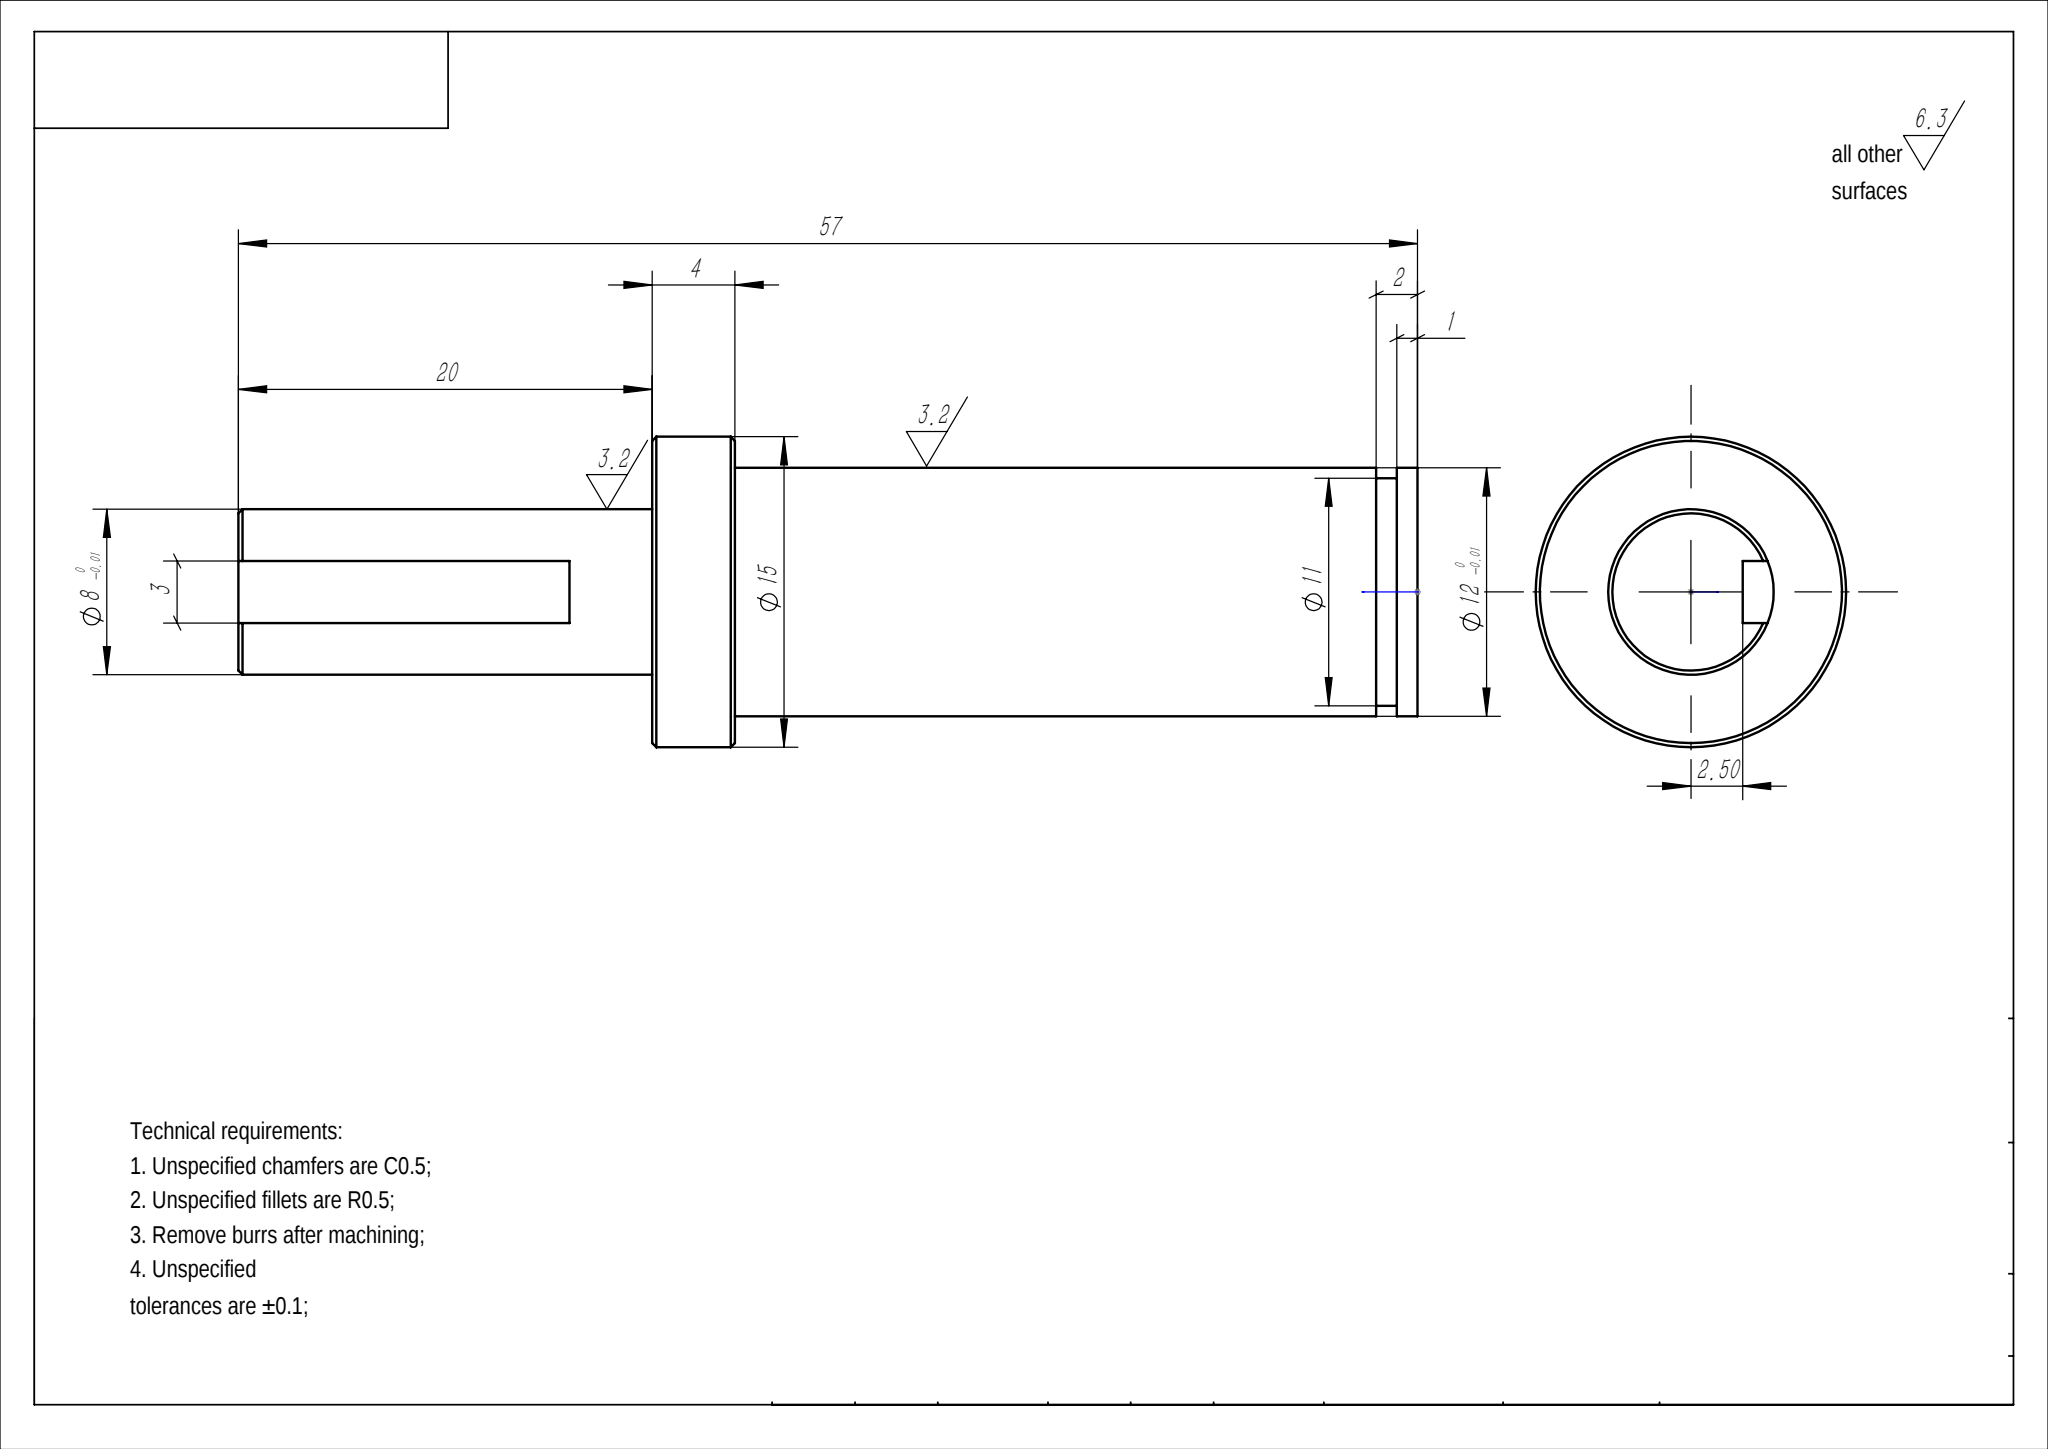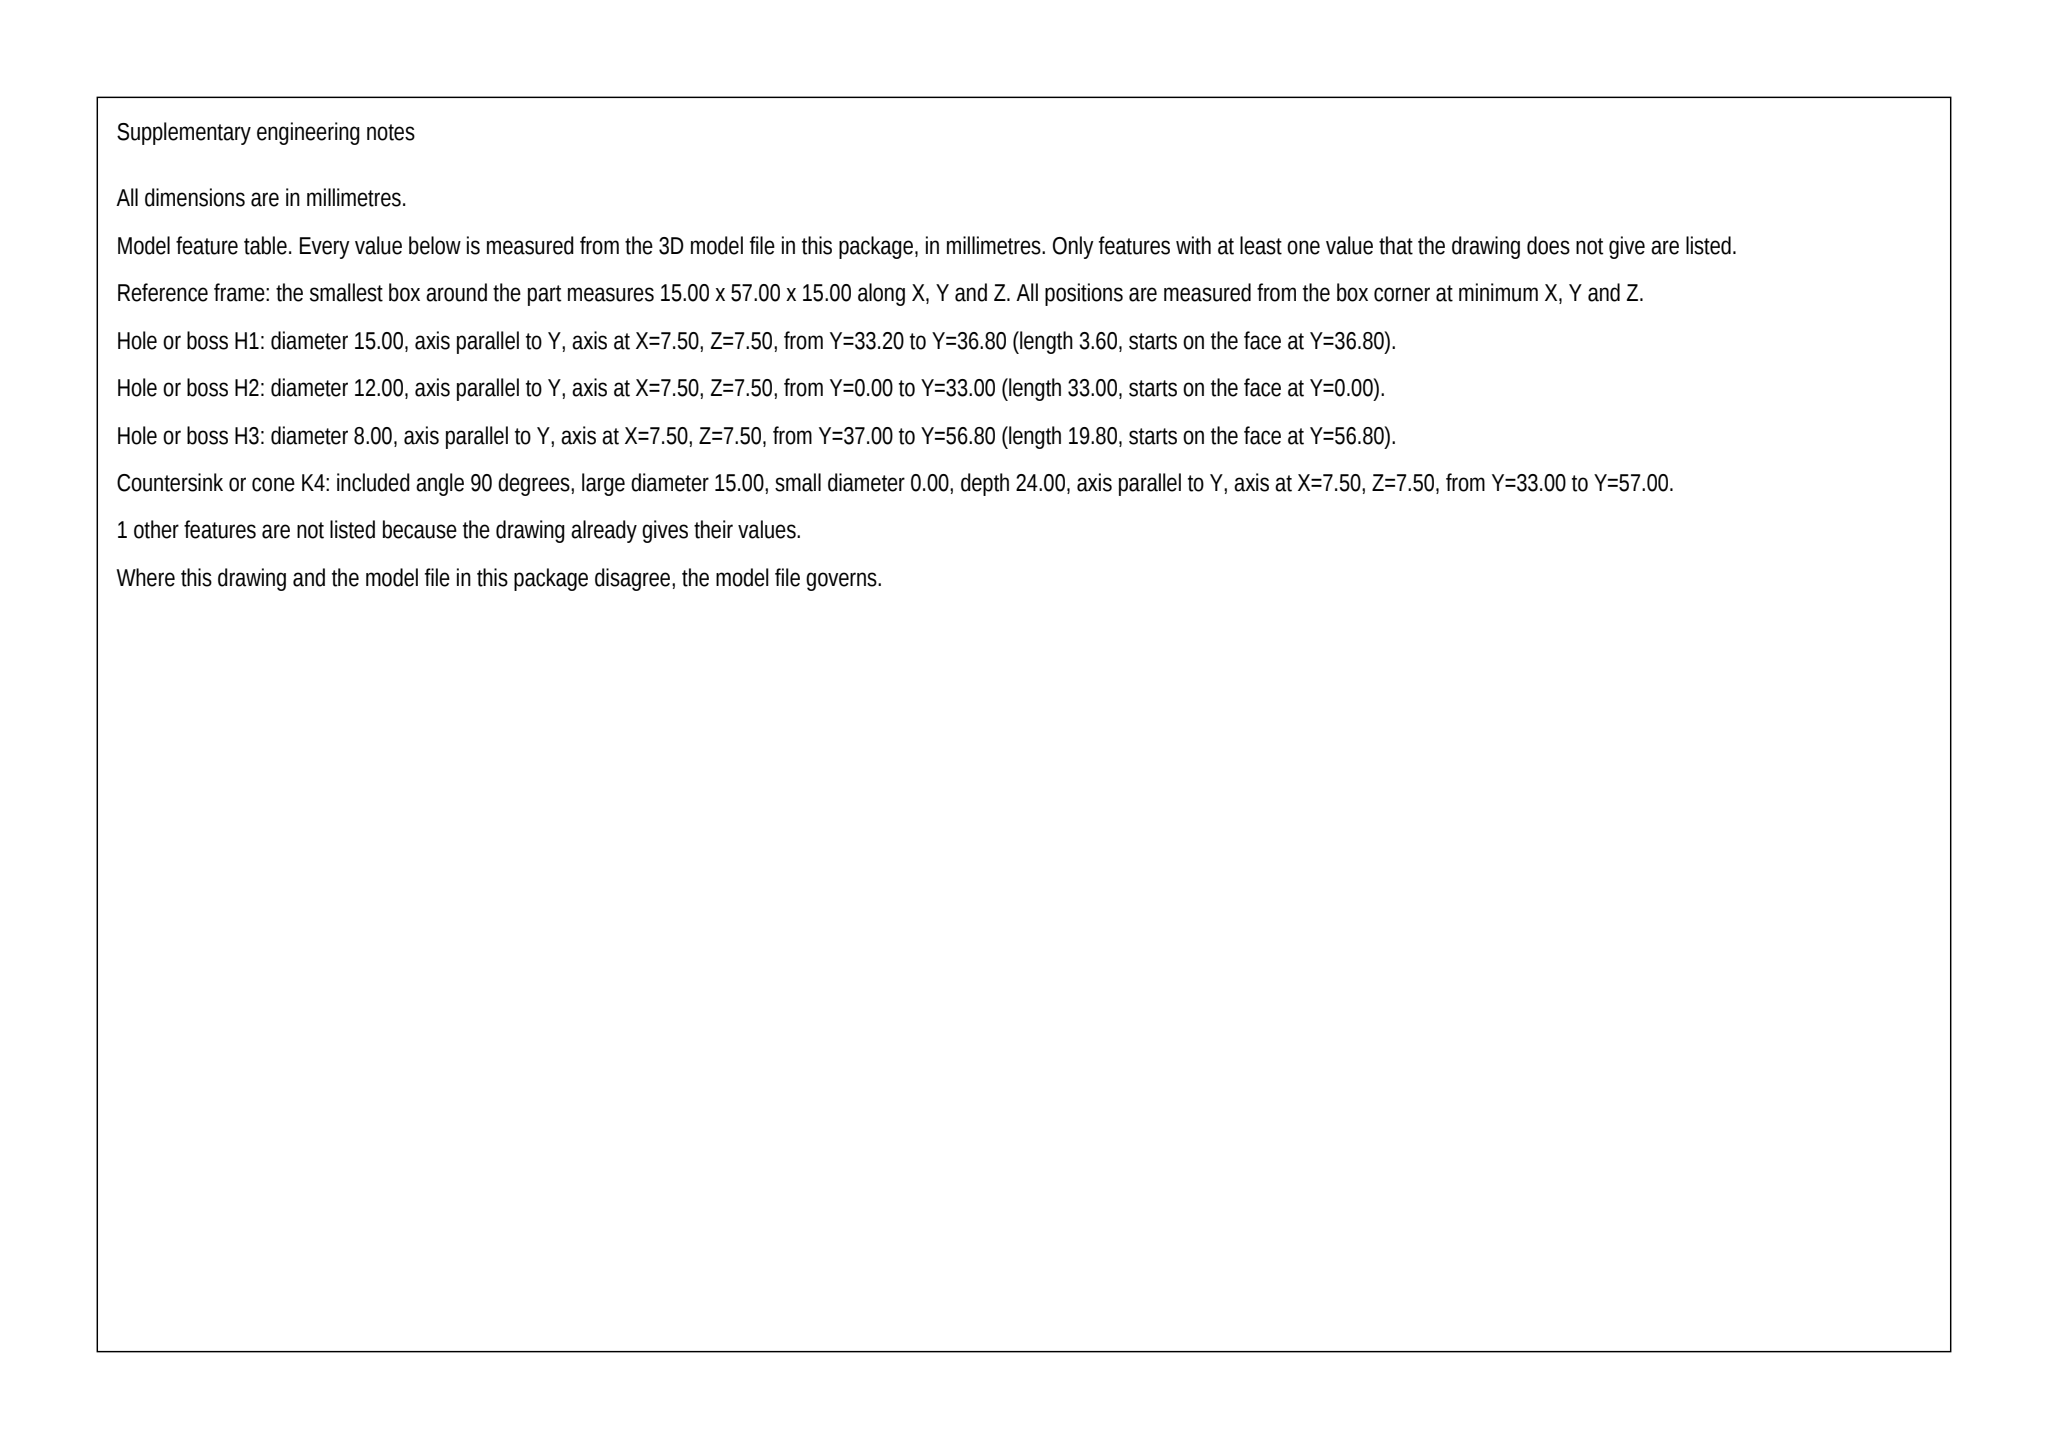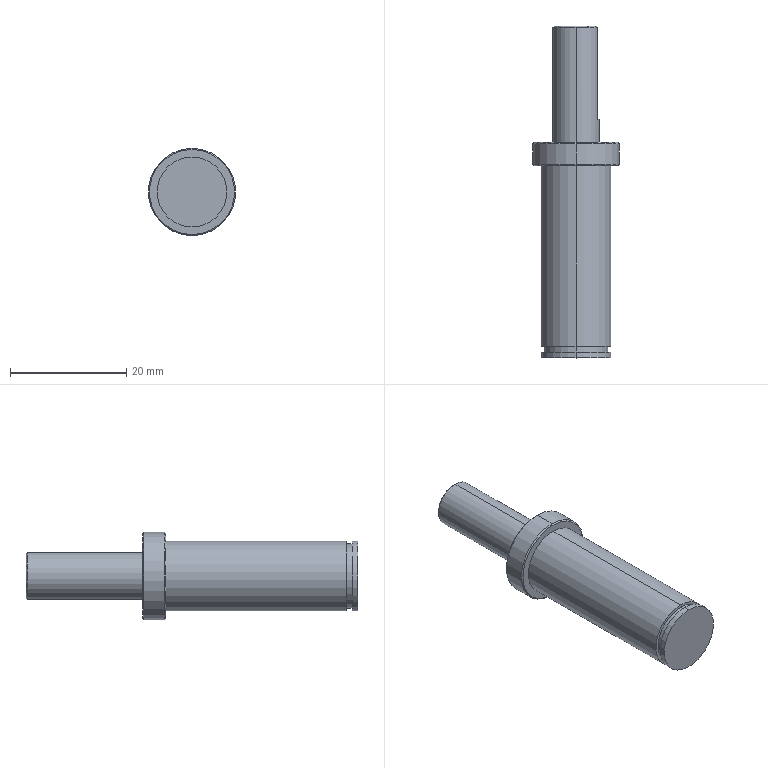Part | SolidWorks | mm | 1 solid | 27 faces | box 15 x 57 x 15 mm | volume 5357 mm3 | cylinder 10 | plane 10 | cone 7 | commonest cylinder face diameters 12 x4 11 x2 8 x2 15 x2
build123d program:
from build123d import *

# Parameters (mm, degrees)
SKETCH1_R           = 6
BOSS_EXTRUDE1_DEPTH = 33
SKETCH2_R           = 7.5
BOSS_EXTRUDE2_DEPTH = 4
SKETCH3_R           = 4
BOSS_EXTRUDE3_DEPTH = 20
SKETCH5_W           = 3
SKETCH5_H           = 3
CUT_EXTRUDE1_DEPTH  = 16
CHAMFER1_SIZE       = 0.2
SKETCH6_W           = 1
SKETCH6_H           = 1


with BuildPart() as part:
    # Sketch1 → Boss-Extrude1 (new body)
    with BuildSketch(Plane(origin=(0, 0, 0), x_dir=(1, 0, 0), z_dir=(0, 1, 0))):
        with Locations(Location((0, 0, 0), (0, 0, 270))):
            Circle(SKETCH1_R)
    extrude(amount=BOSS_EXTRUDE1_DEPTH)

    # Sketch2 → Boss-Extrude2 (add)
    with BuildSketch(Plane(origin=(0, 33, 0), x_dir=(1, 0, 0), z_dir=(0, 1, 0))):
        with Locations(Location((0, 0, 0), (0, 0, 270))):
            Circle(SKETCH2_R)
    extrude(amount=BOSS_EXTRUDE2_DEPTH)

    # Sketch3 → Boss-Extrude3 (add)
    with BuildSketch(Plane(origin=(0, 37, 0), x_dir=(1, 0, 0), z_dir=(0, 1, 0))):
        with Locations(Location((0, 0, 0), (0, 0, 270))):
            Circle(SKETCH3_R)
    extrude(amount=BOSS_EXTRUDE3_DEPTH)

    # Sketch5 → Cut-Extrude1 (cut)
    with BuildSketch(Plane(origin=(0, 57, 0), x_dir=(1, 0, 0), z_dir=(0, 1, 0))):
        with Locations((4, 0)):
            Rectangle(SKETCH5_W, SKETCH5_H)
    extrude(amount=-CUT_EXTRUDE1_DEPTH, mode=Mode.SUBTRACT)

    # Chamfer1
    chamfer1_edges = [part.edges().sort_by_distance(p)[0] for p in [
        (-3.317, 57, -2.236),
        (0, 33, -7.5),
        (0, 37, -7.5),
    ]]
    chamfer(chamfer1_edges, length=CHAMFER1_SIZE)

    # Sketch6 → Cut-Revolve1 (revolve, cut)
    with BuildSketch(Plane.XY, mode=Mode.PRIVATE) as cut_revolve1_sk:
        with Locations((6, 1.5)):
            Rectangle(SKETCH6_W, SKETCH6_H)
    revolve(cut_revolve1_sk.sketch.rotate(Axis((0, 33, 0), (0, -1, 0)), 337.976), axis=Axis((0, 33, 0), (0, -1, 0)), mode=Mode.SUBTRACT)


solid = part.part
STEP:
#1=CARTESIAN_POINT('',(0.,1.,6.));
#2=VERTEX_POINT('',#1);
#3=CARTESIAN_POINT('',(0.,1.,-6.));
#4=VERTEX_POINT('',#3);
#5=CARTESIAN_POINT('',(0.,1.,0.));
#6=DIRECTION('',(0.,1.,0.));
#7=DIRECTION('',(0.,0.,1.));
#8=AXIS2_PLACEMENT_3D('',#5,#6,#7);
#9=CIRCLE('',#8,6.);
#10=EDGE_CURVE('',#2,#4,#9,.T.);
#11=ORIENTED_EDGE('',*,*,#10,.F.);
#12=CARTESIAN_POINT('',(0.,0.,6.));
#13=VERTEX_POINT('',#12);
#14=CARTESIAN_POINT('',(0.,33.,6.));
#15=DIRECTION('',(0.,-1.,0.));
#16=VECTOR('',#15,1000.);
#17=LINE('',#14,#16);
#18=EDGE_CURVE('',#2,#13,#17,.T.);
#19=ORIENTED_EDGE('',*,*,#18,.T.);
#20=CARTESIAN_POINT('',(0.,0.,-6.));
#21=VERTEX_POINT('',#20);
#22=CARTESIAN_POINT('',(0.,0.,0.));
#23=DIRECTION('',(0.,1.,0.));
#24=DIRECTION('',(0.,0.,1.));
#25=AXIS2_PLACEMENT_3D('',#22,#23,#24);
#26=CIRCLE('',#25,6.);
#27=EDGE_CURVE('',#13,#21,#26,.T.);
#28=ORIENTED_EDGE('',*,*,#27,.T.);
#29=CARTESIAN_POINT('',(0.,33.,-6.));
#30=DIRECTION('',(0.,-1.,0.));
#31=VECTOR('',#30,1000.);
#32=LINE('',#29,#31);
#33=EDGE_CURVE('',#4,#21,#32,.T.);
#34=ORIENTED_EDGE('',*,*,#33,.F.);
#35=EDGE_LOOP('',(#11,#19,#28,#34));
#36=FACE_OUTER_BOUND('',#35,.T.);
#37=CARTESIAN_POINT('',(0.,33.,0.));
#38=DIRECTION('',(0.,-1.,0.));
#39=DIRECTION('',(0.,0.,-1.));
#40=AXIS2_PLACEMENT_3D('',#37,#38,#39);
#41=CYLINDRICAL_SURFACE('',#40,6.);
#42=ADVANCED_FACE('',(#36),#41,.T.);
#43=CARTESIAN_POINT('',(0.,1.,5.5));
#44=VERTEX_POINT('',#43);
#45=CARTESIAN_POINT('',(0.,1.,-5.5));
#46=VERTEX_POINT('',#45);
#47=CARTESIAN_POINT('',(0.,1.,0.));
#48=DIRECTION('',(0.,1.,0.));
#49=DIRECTION('',(0.,0.,1.));
#50=AXIS2_PLACEMENT_3D('',#47,#48,#49);
#51=CIRCLE('',#50,5.5);
#52=EDGE_CURVE('',#44,#46,#51,.T.);
#53=ORIENTED_EDGE('',*,*,#52,.T.);
#54=CARTESIAN_POINT('',(0.,2.,-5.5));
#55=VERTEX_POINT('',#54);
#56=CARTESIAN_POINT('',(0.,33.,-5.5));
#57=DIRECTION('',(0.,1.,0.));
#58=VECTOR('',#57,1000.);
#59=LINE('',#56,#58);
#60=EDGE_CURVE('',#46,#55,#59,.T.);
#61=ORIENTED_EDGE('',*,*,#60,.T.);
#62=CARTESIAN_POINT('',(0.,2.,5.5));
#63=VERTEX_POINT('',#62);
#64=CARTESIAN_POINT('',(0.,2.,0.));
#65=DIRECTION('',(0.,1.,0.));
#66=DIRECTION('',(0.,0.,1.));
#67=AXIS2_PLACEMENT_3D('',#64,#65,#66);
#68=CIRCLE('',#67,5.5);
#69=EDGE_CURVE('',#63,#55,#68,.T.);
#70=ORIENTED_EDGE('',*,*,#69,.F.);
#71=CARTESIAN_POINT('',(0.,33.,5.5));
#72=DIRECTION('',(0.,1.,0.));
#73=VECTOR('',#72,1000.);
#74=LINE('',#71,#73);
#75=EDGE_CURVE('',#44,#63,#74,.T.);
#76=ORIENTED_EDGE('',*,*,#75,.F.);
#77=EDGE_LOOP('',(#53,#61,#70,#76));
#78=FACE_OUTER_BOUND('',#77,.T.);
#79=CARTESIAN_POINT('',(0.,33.,0.));
#80=DIRECTION('',(0.,1.,0.));
#81=DIRECTION('',(0.,0.,1.));
#82=AXIS2_PLACEMENT_3D('',#79,#80,#81);
#83=CYLINDRICAL_SURFACE('',#82,5.5);
#84=ADVANCED_FACE('',(#78),#83,.T.);
#85=CARTESIAN_POINT('',(0.,57.,3.8));
#86=VERTEX_POINT('',#85);
#87=CARTESIAN_POINT('',(3.491,57.,1.5));
#88=VERTEX_POINT('',#87);
#89=CARTESIAN_POINT('',(0.,57.,0.));
#90=DIRECTION('',(0.,1.,0.));
#91=DIRECTION('',(0.,0.,1.));
#92=AXIS2_PLACEMENT_3D('',#89,#90,#91);
#93=CIRCLE('',#92,3.8);
#94=EDGE_CURVE('',#86,#88,#93,.T.);
#95=ORIENTED_EDGE('',*,*,#94,.F.);
#96=CARTESIAN_POINT('',(0.,56.8,4.));
#97=VERTEX_POINT('',#96);
#98=CARTESIAN_POINT('',(0.,57.,3.8));
#99=DIRECTION('',(0.,-0.7071,0.7071));
#100=VECTOR('',#99,1000.);
#101=LINE('',#98,#100);
#102=EDGE_CURVE('',#86,#97,#101,.T.);
#103=ORIENTED_EDGE('',*,*,#102,.T.);
#104=CARTESIAN_POINT('',(3.708,56.8,1.5));
#105=VERTEX_POINT('',#104);
#106=CARTESIAN_POINT('',(0.,56.8,0.));
#107=DIRECTION('',(0.,-1.,0.));
#108=DIRECTION('',(-0.,0.,1.));
#109=AXIS2_PLACEMENT_3D('',#106,#107,#108);
#110=CIRCLE('',#109,4.);
#111=EDGE_CURVE('',#105,#97,#110,.T.);
#112=ORIENTED_EDGE('',*,*,#111,.F.);
#113=CARTESIAN_POINT('',(3.491,57.,1.5));
#114=CARTESIAN_POINT('',(3.564,56.933,1.5));
#115=CARTESIAN_POINT('',(3.636,56.867,1.5));
#116=CARTESIAN_POINT('',(3.708,56.8,1.5));
#117=B_SPLINE_CURVE_WITH_KNOTS('',3,(#113,#114,#115,#116),.UNSPECIFIED.,.F.,.F.,(4,4),(0.,0.0002949),.UNSPECIFIED.);
#118=EDGE_CURVE('',#88,#105,#117,.T.);
#119=ORIENTED_EDGE('',*,*,#118,.F.);
#120=EDGE_LOOP('',(#95,#103,#112,#119));
#121=FACE_OUTER_BOUND('',#120,.T.);
#122=CARTESIAN_POINT('',(0.,57.,0.));
#123=DIRECTION('',(0.,-1.,0.));
#124=DIRECTION('',(0.,0.,-1.));
#125=AXIS2_PLACEMENT_3D('',#122,#123,#124);
#126=CONICAL_SURFACE('',#125,3.8,0.7854);
#127=ADVANCED_FACE('',(#121),#126,.T.);
#128=ORIENTED_EDGE('',*,*,#102,.F.);
#129=CARTESIAN_POINT('',(0.,57.,-3.8));
#130=VERTEX_POINT('',#129);
#131=CARTESIAN_POINT('',(0.,57.,0.));
#132=DIRECTION('',(0.,1.,0.));
#133=DIRECTION('',(0.,0.,1.));
#134=AXIS2_PLACEMENT_3D('',#131,#132,#133);
#135=CIRCLE('',#134,3.8);
#136=EDGE_CURVE('',#130,#86,#135,.T.);
#137=ORIENTED_EDGE('',*,*,#136,.F.);
#138=CARTESIAN_POINT('',(0.,56.8,-4.));
#139=VERTEX_POINT('',#138);
#140=CARTESIAN_POINT('',(0.,57.,-3.8));
#141=DIRECTION('',(0.,-0.7071,-0.7071));
#142=VECTOR('',#141,1000.);
#143=LINE('',#140,#142);
#144=EDGE_CURVE('',#130,#139,#143,.T.);
#145=ORIENTED_EDGE('',*,*,#144,.T.);
#146=CARTESIAN_POINT('',(0.,56.8,0.));
#147=DIRECTION('',(0.,-1.,0.));
#148=DIRECTION('',(0.,0.,1.));
#149=AXIS2_PLACEMENT_3D('',#146,#147,#148);
#150=CIRCLE('',#149,4.);
#151=EDGE_CURVE('',#97,#139,#150,.T.);
#152=ORIENTED_EDGE('',*,*,#151,.F.);
#153=EDGE_LOOP('',(#128,#137,#145,#152));
#154=FACE_OUTER_BOUND('',#153,.T.);
#155=CARTESIAN_POINT('',(0.,57.,0.));
#156=DIRECTION('',(0.,-1.,0.));
#157=DIRECTION('',(0.,0.,-1.));
#158=AXIS2_PLACEMENT_3D('',#155,#156,#157);
#159=CONICAL_SURFACE('',#158,3.8,0.7854);
#160=ADVANCED_FACE('',(#154),#159,.T.);
#161=CARTESIAN_POINT('',(0.,37.,7.3));
#162=VERTEX_POINT('',#161);
#163=CARTESIAN_POINT('',(0.,37.,-7.3));
#164=VERTEX_POINT('',#163);
#165=CARTESIAN_POINT('',(0.,37.,0.));
#166=DIRECTION('',(0.,1.,0.));
#167=DIRECTION('',(0.,0.,1.));
#168=AXIS2_PLACEMENT_3D('',#165,#166,#167);
#169=CIRCLE('',#168,7.3);
#170=EDGE_CURVE('',#162,#164,#169,.T.);
#171=ORIENTED_EDGE('',*,*,#170,.F.);
#172=CARTESIAN_POINT('',(0.,36.8,7.5));
#173=VERTEX_POINT('',#172);
#174=CARTESIAN_POINT('',(0.,37.,7.3));
#175=DIRECTION('',(0.,-0.7071,0.7071));
#176=VECTOR('',#175,1000.);
#177=LINE('',#174,#176);
#178=EDGE_CURVE('',#162,#173,#177,.T.);
#179=ORIENTED_EDGE('',*,*,#178,.T.);
#180=CARTESIAN_POINT('',(0.,36.8,-7.5));
#181=VERTEX_POINT('',#180);
#182=CARTESIAN_POINT('',(0.,36.8,0.));
#183=DIRECTION('',(0.,-1.,0.));
#184=DIRECTION('',(0.,0.,1.));
#185=AXIS2_PLACEMENT_3D('',#182,#183,#184);
#186=CIRCLE('',#185,7.5);
#187=EDGE_CURVE('',#181,#173,#186,.T.);
#188=ORIENTED_EDGE('',*,*,#187,.F.);
#189=CARTESIAN_POINT('',(0.,37.,-7.3));
#190=DIRECTION('',(0.,-0.7071,-0.7071));
#191=VECTOR('',#190,1000.);
#192=LINE('',#189,#191);
#193=EDGE_CURVE('',#164,#181,#192,.T.);
#194=ORIENTED_EDGE('',*,*,#193,.F.);
#195=EDGE_LOOP('',(#171,#179,#188,#194));
#196=FACE_OUTER_BOUND('',#195,.T.);
#197=CARTESIAN_POINT('',(0.,37.,0.));
#198=DIRECTION('',(0.,-1.,0.));
#199=DIRECTION('',(0.,0.,-1.));
#200=AXIS2_PLACEMENT_3D('',#197,#198,#199);
#201=CONICAL_SURFACE('',#200,7.3,0.7854);
#202=ADVANCED_FACE('',(#196),#201,.T.);
#203=CARTESIAN_POINT('',(0.,33.,-7.3));
#204=VERTEX_POINT('',#203);
#205=CARTESIAN_POINT('',(0.,33.,7.3));
#206=VERTEX_POINT('',#205);
#207=CARTESIAN_POINT('',(0.,33.,0.));
#208=DIRECTION('',(0.,-1.,0.));
#209=DIRECTION('',(0.,0.,1.));
#210=AXIS2_PLACEMENT_3D('',#207,#208,#209);
#211=CIRCLE('',#210,7.3);
#212=EDGE_CURVE('',#204,#206,#211,.T.);
#213=ORIENTED_EDGE('',*,*,#212,.F.);
#214=CARTESIAN_POINT('',(0.,33.2,-7.5));
#215=VERTEX_POINT('',#214);
#216=CARTESIAN_POINT('',(0.,33.2,-7.5));
#217=DIRECTION('',(0.,0.7071,-0.7071));
#218=VECTOR('',#217,1000.);
#219=LINE('',#216,#218);
#220=EDGE_CURVE('',#204,#215,#219,.T.);
#221=ORIENTED_EDGE('',*,*,#220,.T.);
#222=CARTESIAN_POINT('',(0.,33.2,7.5));
#223=VERTEX_POINT('',#222);
#224=CARTESIAN_POINT('',(0.,33.2,0.));
#225=DIRECTION('',(0.,1.,0.));
#226=DIRECTION('',(0.,0.,1.));
#227=AXIS2_PLACEMENT_3D('',#224,#225,#226);
#228=CIRCLE('',#227,7.5);
#229=EDGE_CURVE('',#223,#215,#228,.T.);
#230=ORIENTED_EDGE('',*,*,#229,.F.);
#231=CARTESIAN_POINT('',(0.,33.2,7.5));
#232=DIRECTION('',(0.,0.7071,0.7071));
#233=VECTOR('',#232,1000.);
#234=LINE('',#231,#233);
#235=EDGE_CURVE('',#206,#223,#234,.T.);
#236=ORIENTED_EDGE('',*,*,#235,.F.);
#237=EDGE_LOOP('',(#213,#221,#230,#236));
#238=FACE_OUTER_BOUND('',#237,.T.);
#239=CARTESIAN_POINT('',(0.,33.2,0.));
#240=DIRECTION('',(0.,1.,0.));
#241=DIRECTION('',(0.,0.,1.));
#242=AXIS2_PLACEMENT_3D('',#239,#240,#241);
#243=CONICAL_SURFACE('',#242,7.5,0.7854);
#244=ADVANCED_FACE('',(#238),#243,.T.);
#245=ORIENTED_EDGE('',*,*,#111,.T.);
#246=CARTESIAN_POINT('',(0.,37.,4.));
#247=VERTEX_POINT('',#246);
#248=CARTESIAN_POINT('',(0.,57.,4.));
#249=DIRECTION('',(0.,-1.,0.));
#250=VECTOR('',#249,1000.);
#251=LINE('',#248,#250);
#252=EDGE_CURVE('',#97,#247,#251,.T.);
#253=ORIENTED_EDGE('',*,*,#252,.T.);
#254=CARTESIAN_POINT('',(0.,37.,-4.));
#255=VERTEX_POINT('',#254);
#256=CARTESIAN_POINT('',(0.,37.,0.));
#257=DIRECTION('',(0.,1.,0.));
#258=DIRECTION('',(0.,0.,1.));
#259=AXIS2_PLACEMENT_3D('',#256,#257,#258);
#260=CIRCLE('',#259,4.);
#261=EDGE_CURVE('',#247,#255,#260,.T.);
#262=ORIENTED_EDGE('',*,*,#261,.T.);
#263=CARTESIAN_POINT('',(0.,57.,-4.));
#264=DIRECTION('',(0.,-1.,0.));
#265=VECTOR('',#264,1000.);
#266=LINE('',#263,#265);
#267=EDGE_CURVE('',#139,#255,#266,.T.);
#268=ORIENTED_EDGE('',*,*,#267,.F.);
#269=CARTESIAN_POINT('',(3.708,56.8,-1.5));
#270=VERTEX_POINT('',#269);
#271=CARTESIAN_POINT('',(0.,56.8,0.));
#272=DIRECTION('',(0.,-1.,0.));
#273=DIRECTION('',(-0.,0.,1.));
#274=AXIS2_PLACEMENT_3D('',#271,#272,#273);
#275=CIRCLE('',#274,4.);
#276=EDGE_CURVE('',#139,#270,#275,.T.);
#277=ORIENTED_EDGE('',*,*,#276,.T.);
#278=CARTESIAN_POINT('',(3.708,41.,-1.5));
#279=VERTEX_POINT('',#278);
#280=CARTESIAN_POINT('',(3.708,57.,-1.5));
#281=DIRECTION('',(0.,-1.,0.));
#282=VECTOR('',#281,1000.);
#283=LINE('',#280,#282);
#284=EDGE_CURVE('',#270,#279,#283,.T.);
#285=ORIENTED_EDGE('',*,*,#284,.T.);
#286=CARTESIAN_POINT('',(3.708,41.,1.5));
#287=VERTEX_POINT('',#286);
#288=CARTESIAN_POINT('',(0.,41.,0.));
#289=DIRECTION('',(0.,1.,0.));
#290=DIRECTION('',(0.,0.,1.));
#291=AXIS2_PLACEMENT_3D('',#288,#289,#290);
#292=CIRCLE('',#291,4.);
#293=EDGE_CURVE('',#287,#279,#292,.T.);
#294=ORIENTED_EDGE('',*,*,#293,.F.);
#295=CARTESIAN_POINT('',(3.708,57.,1.5));
#296=DIRECTION('',(0.,1.,0.));
#297=VECTOR('',#296,1000.);
#298=LINE('',#295,#297);
#299=EDGE_CURVE('',#287,#105,#298,.T.);
#300=ORIENTED_EDGE('',*,*,#299,.T.);
#301=EDGE_LOOP('',(#245,#253,#262,#268,#277,#285,#294,#300));
#302=FACE_OUTER_BOUND('',#301,.T.);
#303=CARTESIAN_POINT('',(0.,57.,0.));
#304=DIRECTION('',(0.,-1.,0.));
#305=DIRECTION('',(0.,0.,-1.));
#306=AXIS2_PLACEMENT_3D('',#303,#304,#305);
#307=CYLINDRICAL_SURFACE('',#306,4.);
#308=ADVANCED_FACE('',(#302),#307,.T.);
#309=ORIENTED_EDGE('',*,*,#187,.T.);
#310=CARTESIAN_POINT('',(0.,37.,7.5));
#311=DIRECTION('',(0.,-1.,0.));
#312=VECTOR('',#311,1000.);
#313=LINE('',#310,#312);
#314=EDGE_CURVE('',#173,#223,#313,.T.);
#315=ORIENTED_EDGE('',*,*,#314,.T.);
#316=ORIENTED_EDGE('',*,*,#229,.T.);
#317=CARTESIAN_POINT('',(0.,37.,-7.5));
#318=DIRECTION('',(0.,-1.,0.));
#319=VECTOR('',#318,1000.);
#320=LINE('',#317,#319);
#321=EDGE_CURVE('',#181,#215,#320,.T.);
#322=ORIENTED_EDGE('',*,*,#321,.F.);
#323=EDGE_LOOP('',(#309,#315,#316,#322));
#324=FACE_OUTER_BOUND('',#323,.T.);
#325=CARTESIAN_POINT('',(0.,37.,0.));
#326=DIRECTION('',(0.,-1.,0.));
#327=DIRECTION('',(0.,0.,-1.));
#328=AXIS2_PLACEMENT_3D('',#325,#326,#327);
#329=CYLINDRICAL_SURFACE('',#328,7.5);
#330=ADVANCED_FACE('',(#324),#329,.T.);
#331=CARTESIAN_POINT('',(0.,33.,6.));
#332=VERTEX_POINT('',#331);
#333=CARTESIAN_POINT('',(0.,33.,-6.));
#334=VERTEX_POINT('',#333);
#335=CARTESIAN_POINT('',(0.,33.,0.));
#336=DIRECTION('',(0.,1.,0.));
#337=DIRECTION('',(0.,0.,1.));
#338=AXIS2_PLACEMENT_3D('',#335,#336,#337);
#339=CIRCLE('',#338,6.);
#340=EDGE_CURVE('',#332,#334,#339,.T.);
#341=ORIENTED_EDGE('',*,*,#340,.F.);
#342=CARTESIAN_POINT('',(0.,2.,6.));
#343=VERTEX_POINT('',#342);
#344=CARTESIAN_POINT('',(0.,33.,6.));
#345=DIRECTION('',(0.,-1.,0.));
#346=VECTOR('',#345,1000.);
#347=LINE('',#344,#346);
#348=EDGE_CURVE('',#332,#343,#347,.T.);
#349=ORIENTED_EDGE('',*,*,#348,.T.);
#350=CARTESIAN_POINT('',(0.,2.,-6.));
#351=VERTEX_POINT('',#350);
#352=CARTESIAN_POINT('',(0.,2.,0.));
#353=DIRECTION('',(0.,-1.,0.));
#354=DIRECTION('',(0.,0.,-1.));
#355=AXIS2_PLACEMENT_3D('',#352,#353,#354);
#356=CIRCLE('',#355,6.);
#357=EDGE_CURVE('',#351,#343,#356,.T.);
#358=ORIENTED_EDGE('',*,*,#357,.F.);
#359=CARTESIAN_POINT('',(0.,33.,-6.));
#360=DIRECTION('',(0.,-1.,0.));
#361=VECTOR('',#360,1000.);
#362=LINE('',#359,#361);
#363=EDGE_CURVE('',#334,#351,#362,.T.);
#364=ORIENTED_EDGE('',*,*,#363,.F.);
#365=EDGE_LOOP('',(#341,#349,#358,#364));
#366=FACE_OUTER_BOUND('',#365,.T.);
#367=CARTESIAN_POINT('',(0.,33.,0.));
#368=DIRECTION('',(0.,-1.,0.));
#369=DIRECTION('',(0.,0.,-1.));
#370=AXIS2_PLACEMENT_3D('',#367,#368,#369);
#371=CYLINDRICAL_SURFACE('',#370,6.);
#372=ADVANCED_FACE('',(#366),#371,.T.);
#373=ORIENTED_EDGE('',*,*,#348,.F.);
#374=CARTESIAN_POINT('',(0.,33.,0.));
#375=DIRECTION('',(0.,1.,0.));
#376=DIRECTION('',(0.,0.,1.));
#377=AXIS2_PLACEMENT_3D('',#374,#375,#376);
#378=CIRCLE('',#377,6.);
#379=EDGE_CURVE('',#334,#332,#378,.T.);
#380=ORIENTED_EDGE('',*,*,#379,.F.);
#381=ORIENTED_EDGE('',*,*,#363,.T.);
#382=CARTESIAN_POINT('',(0.,2.,0.));
#383=DIRECTION('',(0.,-1.,0.));
#384=DIRECTION('',(0.,0.,-1.));
#385=AXIS2_PLACEMENT_3D('',#382,#383,#384);
#386=CIRCLE('',#385,6.);
#387=EDGE_CURVE('',#343,#351,#386,.T.);
#388=ORIENTED_EDGE('',*,*,#387,.F.);
#389=EDGE_LOOP('',(#373,#380,#381,#388));
#390=FACE_OUTER_BOUND('',#389,.T.);
#391=CARTESIAN_POINT('',(0.,33.,0.));
#392=DIRECTION('',(0.,-1.,0.));
#393=DIRECTION('',(0.,0.,-1.));
#394=AXIS2_PLACEMENT_3D('',#391,#392,#393);
#395=CYLINDRICAL_SURFACE('',#394,6.);
#396=ADVANCED_FACE('',(#390),#395,.T.);
#397=CARTESIAN_POINT('',(0.,37.,0.));
#398=DIRECTION('',(0.,1.,0.));
#399=DIRECTION('',(0.,0.,1.));
#400=AXIS2_PLACEMENT_3D('',#397,#398,#399);
#401=CIRCLE('',#400,7.3);
#402=EDGE_CURVE('',#164,#162,#401,.T.);
#403=ORIENTED_EDGE('',*,*,#402,.T.);
#404=ORIENTED_EDGE('',*,*,#170,.T.);
#405=EDGE_LOOP('',(#403,#404));
#406=FACE_OUTER_BOUND('',#405,.T.);
#407=CARTESIAN_POINT('',(0.,37.,0.));
#408=DIRECTION('',(0.,1.,0.));
#409=DIRECTION('',(0.,0.,1.));
#410=AXIS2_PLACEMENT_3D('',#407,#408,#409);
#411=CIRCLE('',#410,4.);
#412=EDGE_CURVE('',#255,#247,#411,.T.);
#413=ORIENTED_EDGE('',*,*,#412,.F.);
#414=ORIENTED_EDGE('',*,*,#261,.F.);
#415=EDGE_LOOP('',(#413,#414));
#416=FACE_BOUND('',#415,.T.);
#417=CARTESIAN_POINT('',(0.,37.,0.));
#418=DIRECTION('',(0.,1.,0.));
#419=DIRECTION('',(0.,0.,1.));
#420=AXIS2_PLACEMENT_3D('',#417,#418,#419);
#421=PLANE('',#420);
#422=ADVANCED_FACE('',(#406,#416),#421,.T.);
#423=CARTESIAN_POINT('',(0.,33.,0.));
#424=DIRECTION('',(0.,-1.,0.));
#425=DIRECTION('',(0.,0.,1.));
#426=AXIS2_PLACEMENT_3D('',#423,#424,#425);
#427=CIRCLE('',#426,7.3);
#428=EDGE_CURVE('',#206,#204,#427,.T.);
#429=ORIENTED_EDGE('',*,*,#428,.T.);
#430=ORIENTED_EDGE('',*,*,#212,.T.);
#431=EDGE_LOOP('',(#429,#430));
#432=FACE_OUTER_BOUND('',#431,.T.);
#433=ORIENTED_EDGE('',*,*,#379,.T.);
#434=ORIENTED_EDGE('',*,*,#340,.T.);
#435=EDGE_LOOP('',(#433,#434));
#436=FACE_BOUND('',#435,.T.);
#437=CARTESIAN_POINT('',(0.,33.,0.));
#438=DIRECTION('',(0.,1.,0.));
#439=DIRECTION('',(0.,0.,1.));
#440=AXIS2_PLACEMENT_3D('',#437,#438,#439);
#441=PLANE('',#440);
#442=ADVANCED_FACE('',(#432,#436),#441,.F.);
#443=ORIENTED_EDGE('',*,*,#314,.F.);
#444=CARTESIAN_POINT('',(0.,36.8,0.));
#445=DIRECTION('',(0.,-1.,0.));
#446=DIRECTION('',(0.,0.,1.));
#447=AXIS2_PLACEMENT_3D('',#444,#445,#446);
#448=CIRCLE('',#447,7.5);
#449=EDGE_CURVE('',#173,#181,#448,.T.);
#450=ORIENTED_EDGE('',*,*,#449,.T.);
#451=ORIENTED_EDGE('',*,*,#321,.T.);
#452=CARTESIAN_POINT('',(0.,33.2,0.));
#453=DIRECTION('',(0.,1.,0.));
#454=DIRECTION('',(0.,0.,1.));
#455=AXIS2_PLACEMENT_3D('',#452,#453,#454);
#456=CIRCLE('',#455,7.5);
#457=EDGE_CURVE('',#215,#223,#456,.T.);
#458=ORIENTED_EDGE('',*,*,#457,.T.);
#459=EDGE_LOOP('',(#443,#450,#451,#458));
#460=FACE_OUTER_BOUND('',#459,.T.);
#461=CARTESIAN_POINT('',(0.,37.,0.));
#462=DIRECTION('',(0.,-1.,0.));
#463=DIRECTION('',(0.,0.,-1.));
#464=AXIS2_PLACEMENT_3D('',#461,#462,#463);
#465=CYLINDRICAL_SURFACE('',#464,7.5);
#466=ADVANCED_FACE('',(#460),#465,.T.);
#467=ORIENTED_EDGE('',*,*,#252,.F.);
#468=ORIENTED_EDGE('',*,*,#151,.T.);
#469=ORIENTED_EDGE('',*,*,#267,.T.);
#470=ORIENTED_EDGE('',*,*,#412,.T.);
#471=EDGE_LOOP('',(#467,#468,#469,#470));
#472=FACE_OUTER_BOUND('',#471,.T.);
#473=CARTESIAN_POINT('',(0.,57.,0.));
#474=DIRECTION('',(0.,-1.,0.));
#475=DIRECTION('',(0.,0.,-1.));
#476=AXIS2_PLACEMENT_3D('',#473,#474,#475);
#477=CYLINDRICAL_SURFACE('',#476,4.);
#478=ADVANCED_FACE('',(#472),#477,.T.);
#479=CARTESIAN_POINT('',(3.491,57.,-1.5));
#480=VERTEX_POINT('',#479);
#481=CARTESIAN_POINT('',(2.5,57.,-1.5));
#482=VERTEX_POINT('',#481);
#483=CARTESIAN_POINT('',(0.,57.,-1.5));
#484=DIRECTION('',(-1.,0.,0.));
#485=VECTOR('',#484,1000.);
#486=LINE('',#483,#485);
#487=EDGE_CURVE('',#480,#482,#486,.T.);
#488=ORIENTED_EDGE('',*,*,#487,.F.);
#489=CARTESIAN_POINT('',(0.,57.,0.));
#490=DIRECTION('',(0.,1.,0.));
#491=DIRECTION('',(0.,0.,1.));
#492=AXIS2_PLACEMENT_3D('',#489,#490,#491);
#493=CIRCLE('',#492,3.8);
#494=EDGE_CURVE('',#480,#130,#493,.T.);
#495=ORIENTED_EDGE('',*,*,#494,.T.);
#496=ORIENTED_EDGE('',*,*,#136,.T.);
#497=ORIENTED_EDGE('',*,*,#94,.T.);
#498=CARTESIAN_POINT('',(2.5,57.,1.5));
#499=VERTEX_POINT('',#498);
#500=CARTESIAN_POINT('',(2.5,57.,1.5));
#501=DIRECTION('',(1.,0.,0.));
#502=VECTOR('',#501,1000.);
#503=LINE('',#500,#502);
#504=EDGE_CURVE('',#499,#88,#503,.T.);
#505=ORIENTED_EDGE('',*,*,#504,.F.);
#506=CARTESIAN_POINT('',(2.5,57.,-1.5));
#507=DIRECTION('',(0.,0.,1.));
#508=VECTOR('',#507,1000.);
#509=LINE('',#506,#508);
#510=EDGE_CURVE('',#482,#499,#509,.T.);
#511=ORIENTED_EDGE('',*,*,#510,.F.);
#512=EDGE_LOOP('',(#488,#495,#496,#497,#505,#511));
#513=FACE_OUTER_BOUND('',#512,.T.);
#514=CARTESIAN_POINT('',(0.,57.,0.));
#515=DIRECTION('',(0.,1.,0.));
#516=DIRECTION('',(0.,0.,1.));
#517=AXIS2_PLACEMENT_3D('',#514,#515,#516);
#518=PLANE('',#517);
#519=ADVANCED_FACE('',(#513),#518,.T.);
#520=ORIENTED_EDGE('',*,*,#293,.T.);
#521=CARTESIAN_POINT('',(2.5,41.,-1.5));
#522=VERTEX_POINT('',#521);
#523=CARTESIAN_POINT('',(2.5,41.,-1.5));
#524=DIRECTION('',(-1.,0.,0.));
#525=VECTOR('',#524,1000.);
#526=LINE('',#523,#525);
#527=EDGE_CURVE('',#279,#522,#526,.T.);
#528=ORIENTED_EDGE('',*,*,#527,.T.);
#529=CARTESIAN_POINT('',(2.5,41.,1.5));
#530=VERTEX_POINT('',#529);
#531=CARTESIAN_POINT('',(2.5,41.,-1.5));
#532=DIRECTION('',(0.,0.,1.));
#533=VECTOR('',#532,1000.);
#534=LINE('',#531,#533);
#535=EDGE_CURVE('',#522,#530,#534,.T.);
#536=ORIENTED_EDGE('',*,*,#535,.T.);
#537=CARTESIAN_POINT('',(2.5,41.,1.5));
#538=DIRECTION('',(1.,0.,0.));
#539=VECTOR('',#538,1000.);
#540=LINE('',#537,#539);
#541=EDGE_CURVE('',#530,#287,#540,.T.);
#542=ORIENTED_EDGE('',*,*,#541,.T.);
#543=EDGE_LOOP('',(#520,#528,#536,#542));
#544=FACE_OUTER_BOUND('',#543,.T.);
#545=CARTESIAN_POINT('',(0.,41.,0.));
#546=DIRECTION('',(0.,1.,0.));
#547=DIRECTION('',(0.,0.,1.));
#548=AXIS2_PLACEMENT_3D('',#545,#546,#547);
#549=PLANE('',#548);
#550=ADVANCED_FACE('',(#544),#549,.T.);
#551=ORIENTED_EDGE('',*,*,#504,.T.);
#552=ORIENTED_EDGE('',*,*,#118,.T.);
#553=ORIENTED_EDGE('',*,*,#299,.F.);
#554=ORIENTED_EDGE('',*,*,#541,.F.);
#555=CARTESIAN_POINT('',(2.5,41.,1.5));
#556=DIRECTION('',(0.,1.,0.));
#557=VECTOR('',#556,1000.);
#558=LINE('',#555,#557);
#559=EDGE_CURVE('',#530,#499,#558,.T.);
#560=ORIENTED_EDGE('',*,*,#559,.T.);
#561=EDGE_LOOP('',(#551,#552,#553,#554,#560));
#562=FACE_OUTER_BOUND('',#561,.T.);
#563=CARTESIAN_POINT('',(2.5,41.,1.5));
#564=DIRECTION('',(0.,0.,1.));
#565=DIRECTION('',(1.,0.,0.));
#566=AXIS2_PLACEMENT_3D('',#563,#564,#565);
#567=PLANE('',#566);
#568=ADVANCED_FACE('',(#562),#567,.F.);
#569=ORIENTED_EDGE('',*,*,#284,.F.);
#570=CARTESIAN_POINT('',(3.708,56.8,-1.5));
#571=CARTESIAN_POINT('',(3.636,56.867,-1.5));
#572=CARTESIAN_POINT('',(3.564,56.933,-1.5));
#573=CARTESIAN_POINT('',(3.491,57.,-1.5));
#574=B_SPLINE_CURVE_WITH_KNOTS('',3,(#570,#571,#572,#573),.UNSPECIFIED.,.F.,.F.,(4,4),(0.,0.0002949),.UNSPECIFIED.);
#575=EDGE_CURVE('',#270,#480,#574,.T.);
#576=ORIENTED_EDGE('',*,*,#575,.T.);
#577=ORIENTED_EDGE('',*,*,#487,.T.);
#578=CARTESIAN_POINT('',(2.5,41.,-1.5));
#579=DIRECTION('',(0.,1.,0.));
#580=VECTOR('',#579,1000.);
#581=LINE('',#578,#580);
#582=EDGE_CURVE('',#522,#482,#581,.T.);
#583=ORIENTED_EDGE('',*,*,#582,.F.);
#584=ORIENTED_EDGE('',*,*,#527,.F.);
#585=EDGE_LOOP('',(#569,#576,#577,#583,#584));
#586=FACE_OUTER_BOUND('',#585,.T.);
#587=CARTESIAN_POINT('',(2.5,41.,-1.5));
#588=DIRECTION('',(0.,0.,-1.));
#589=DIRECTION('',(-1.,0.,0.));
#590=AXIS2_PLACEMENT_3D('',#587,#588,#589);
#591=PLANE('',#590);
#592=ADVANCED_FACE('',(#586),#591,.F.);
#593=ORIENTED_EDGE('',*,*,#510,.T.);
#594=ORIENTED_EDGE('',*,*,#559,.F.);
#595=ORIENTED_EDGE('',*,*,#535,.F.);
#596=ORIENTED_EDGE('',*,*,#582,.T.);
#597=EDGE_LOOP('',(#593,#594,#595,#596));
#598=FACE_OUTER_BOUND('',#597,.T.);
#599=CARTESIAN_POINT('',(2.5,41.,-1.5));
#600=DIRECTION('',(-1.,0.,0.));
#601=DIRECTION('',(0.,0.,1.));
#602=AXIS2_PLACEMENT_3D('',#599,#600,#601);
#603=PLANE('',#602);
#604=ADVANCED_FACE('',(#598),#603,.F.);
#605=ORIENTED_EDGE('',*,*,#220,.F.);
#606=ORIENTED_EDGE('',*,*,#428,.F.);
#607=ORIENTED_EDGE('',*,*,#235,.T.);
#608=ORIENTED_EDGE('',*,*,#457,.F.);
#609=EDGE_LOOP('',(#605,#606,#607,#608));
#610=FACE_OUTER_BOUND('',#609,.T.);
#611=CARTESIAN_POINT('',(0.,33.2,0.));
#612=DIRECTION('',(0.,1.,0.));
#613=DIRECTION('',(0.,0.,1.));
#614=AXIS2_PLACEMENT_3D('',#611,#612,#613);
#615=CONICAL_SURFACE('',#614,7.5,0.7854);
#616=ADVANCED_FACE('',(#610),#615,.T.);
#617=ORIENTED_EDGE('',*,*,#178,.F.);
#618=ORIENTED_EDGE('',*,*,#402,.F.);
#619=ORIENTED_EDGE('',*,*,#193,.T.);
#620=ORIENTED_EDGE('',*,*,#449,.F.);
#621=EDGE_LOOP('',(#617,#618,#619,#620));
#622=FACE_OUTER_BOUND('',#621,.T.);
#623=CARTESIAN_POINT('',(0.,37.,0.));
#624=DIRECTION('',(0.,-1.,0.));
#625=DIRECTION('',(0.,0.,-1.));
#626=AXIS2_PLACEMENT_3D('',#623,#624,#625);
#627=CONICAL_SURFACE('',#626,7.3,0.7854);
#628=ADVANCED_FACE('',(#622),#627,.T.);
#629=ORIENTED_EDGE('',*,*,#144,.F.);
#630=ORIENTED_EDGE('',*,*,#494,.F.);
#631=ORIENTED_EDGE('',*,*,#575,.F.);
#632=ORIENTED_EDGE('',*,*,#276,.F.);
#633=EDGE_LOOP('',(#629,#630,#631,#632));
#634=FACE_OUTER_BOUND('',#633,.T.);
#635=CARTESIAN_POINT('',(0.,57.,0.));
#636=DIRECTION('',(0.,-1.,0.));
#637=DIRECTION('',(0.,0.,-1.));
#638=AXIS2_PLACEMENT_3D('',#635,#636,#637);
#639=CONICAL_SURFACE('',#638,3.8,0.7854);
#640=ADVANCED_FACE('',(#634),#639,.T.);
#641=ORIENTED_EDGE('',*,*,#69,.T.);
#642=CARTESIAN_POINT('',(0.,2.,0.));
#643=DIRECTION('',(0.,1.,0.));
#644=DIRECTION('',(0.,0.,1.));
#645=AXIS2_PLACEMENT_3D('',#642,#643,#644);
#646=CIRCLE('',#645,5.5);
#647=EDGE_CURVE('',#55,#63,#646,.T.);
#648=ORIENTED_EDGE('',*,*,#647,.T.);
#649=EDGE_LOOP('',(#641,#648));
#650=FACE_BOUND('',#649,.T.);
#651=ORIENTED_EDGE('',*,*,#357,.T.);
#652=ORIENTED_EDGE('',*,*,#387,.T.);
#653=EDGE_LOOP('',(#651,#652));
#654=FACE_OUTER_BOUND('',#653,.T.);
#655=CARTESIAN_POINT('',(5.5,2.,0.));
#656=DIRECTION('',(0.,-1.,0.));
#657=DIRECTION('',(0.,0.,-1.));
#658=AXIS2_PLACEMENT_3D('',#655,#656,#657);
#659=PLANE('',#658);
#660=ADVANCED_FACE('',(#650,#654),#659,.T.);
#661=ORIENTED_EDGE('',*,*,#52,.F.);
#662=CARTESIAN_POINT('',(0.,1.,0.));
#663=DIRECTION('',(0.,1.,0.));
#664=DIRECTION('',(0.,0.,1.));
#665=AXIS2_PLACEMENT_3D('',#662,#663,#664);
#666=CIRCLE('',#665,5.5);
#667=EDGE_CURVE('',#46,#44,#666,.T.);
#668=ORIENTED_EDGE('',*,*,#667,.F.);
#669=EDGE_LOOP('',(#661,#668));
#670=FACE_BOUND('',#669,.T.);
#671=CARTESIAN_POINT('',(0.,1.,0.));
#672=DIRECTION('',(0.,1.,0.));
#673=DIRECTION('',(0.,0.,1.));
#674=AXIS2_PLACEMENT_3D('',#671,#672,#673);
#675=CIRCLE('',#674,6.);
#676=EDGE_CURVE('',#4,#2,#675,.T.);
#677=ORIENTED_EDGE('',*,*,#676,.T.);
#678=ORIENTED_EDGE('',*,*,#10,.T.);
#679=EDGE_LOOP('',(#677,#678));
#680=FACE_OUTER_BOUND('',#679,.T.);
#681=CARTESIAN_POINT('',(5.5,1.,0.));
#682=DIRECTION('',(0.,1.,0.));
#683=DIRECTION('',(0.,0.,1.));
#684=AXIS2_PLACEMENT_3D('',#681,#682,#683);
#685=PLANE('',#684);
#686=ADVANCED_FACE('',(#670,#680),#685,.T.);
#687=ORIENTED_EDGE('',*,*,#60,.F.);
#688=ORIENTED_EDGE('',*,*,#667,.T.);
#689=ORIENTED_EDGE('',*,*,#75,.T.);
#690=ORIENTED_EDGE('',*,*,#647,.F.);
#691=EDGE_LOOP('',(#687,#688,#689,#690));
#692=FACE_OUTER_BOUND('',#691,.T.);
#693=CARTESIAN_POINT('',(0.,33.,0.));
#694=DIRECTION('',(0.,1.,0.));
#695=DIRECTION('',(0.,0.,1.));
#696=AXIS2_PLACEMENT_3D('',#693,#694,#695);
#697=CYLINDRICAL_SURFACE('',#696,5.5);
#698=ADVANCED_FACE('',(#692),#697,.T.);
#699=CARTESIAN_POINT('',(0.,0.,0.));
#700=DIRECTION('',(0.,1.,0.));
#701=DIRECTION('',(0.,0.,1.));
#702=AXIS2_PLACEMENT_3D('',#699,#700,#701);
#703=CIRCLE('',#702,6.);
#704=EDGE_CURVE('',#21,#13,#703,.T.);
#705=ORIENTED_EDGE('',*,*,#704,.F.);
#706=ORIENTED_EDGE('',*,*,#27,.F.);
#707=EDGE_LOOP('',(#705,#706));
#708=FACE_OUTER_BOUND('',#707,.T.);
#709=CARTESIAN_POINT('',(0.,0.,0.));
#710=DIRECTION('',(0.,1.,0.));
#711=DIRECTION('',(0.,0.,1.));
#712=AXIS2_PLACEMENT_3D('',#709,#710,#711);
#713=PLANE('',#712);
#714=ADVANCED_FACE('',(#708),#713,.F.);
#715=ORIENTED_EDGE('',*,*,#18,.F.);
#716=ORIENTED_EDGE('',*,*,#676,.F.);
#717=ORIENTED_EDGE('',*,*,#33,.T.);
#718=ORIENTED_EDGE('',*,*,#704,.T.);
#719=EDGE_LOOP('',(#715,#716,#717,#718));
#720=FACE_OUTER_BOUND('',#719,.T.);
#721=CARTESIAN_POINT('',(0.,33.,0.));
#722=DIRECTION('',(0.,-1.,0.));
#723=DIRECTION('',(0.,0.,-1.));
#724=AXIS2_PLACEMENT_3D('',#721,#722,#723);
#725=CYLINDRICAL_SURFACE('',#724,6.);
#726=ADVANCED_FACE('',(#720),#725,.T.);
#727=CLOSED_SHELL('',(#42,#84,#127,#160,#202,#244,#308,#330,#372,#396,#422,#442,#466,#478,#519,#550,#568,#592,#604,#616,#628,#640,#660,#686,#698,#714,#726));
#728=MANIFOLD_SOLID_BREP('',#727);
#729=CARTESIAN_POINT('',(0.,0.,0.));
#730=DIRECTION('',(0.,0.,1.));
#731=DIRECTION('',(1.,0.,0.));
#732=AXIS2_PLACEMENT_3D('',#729,#730,#731);
#733=(LENGTH_UNIT()NAMED_UNIT(*)SI_UNIT(.MILLI.,.METRE.));
#734=UNCERTAINTY_MEASURE_WITH_UNIT(LENGTH_MEASURE(0.00001),#733,'','');
#735=(NAMED_UNIT(*)PLANE_ANGLE_UNIT()SI_UNIT($,.RADIAN.));
#736=(NAMED_UNIT(*)SI_UNIT($,.STERADIAN.)SOLID_ANGLE_UNIT());
#737=(GEOMETRIC_REPRESENTATION_CONTEXT(3)GLOBAL_UNCERTAINTY_ASSIGNED_CONTEXT((#734))GLOBAL_UNIT_ASSIGNED_CONTEXT((#733,#735,#736))REPRESENTATION_CONTEXT('',''));
#738=ADVANCED_BREP_SHAPE_REPRESENTATION('',(#728,#732),#737);